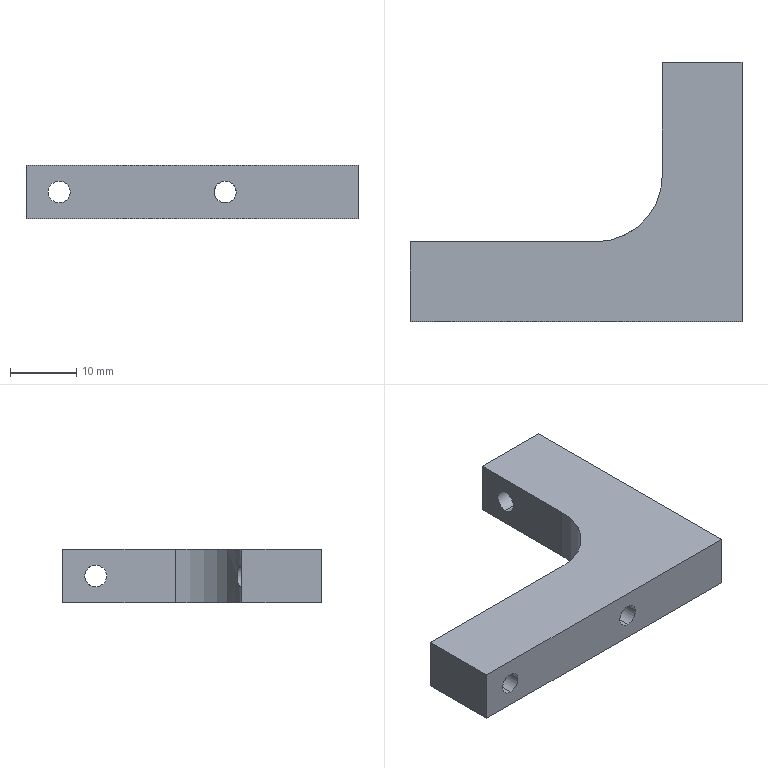CAM job | Mastercam | mm | 4 operations | part box 50 x 39 x 8
1. Drill/Counterbore | 2 - 6定位倒角
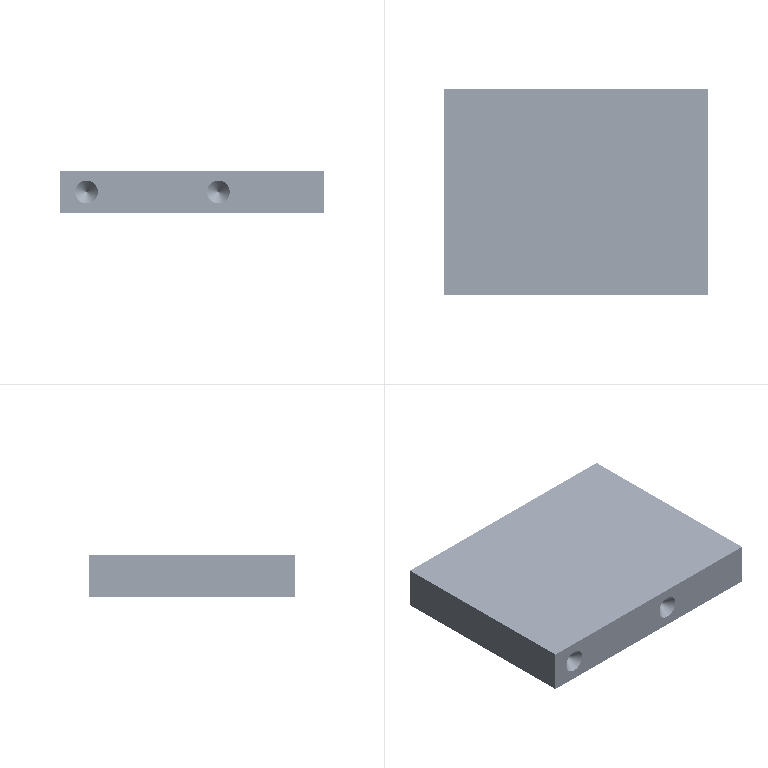2. Peck Drill | 12 - 3.3 钻头
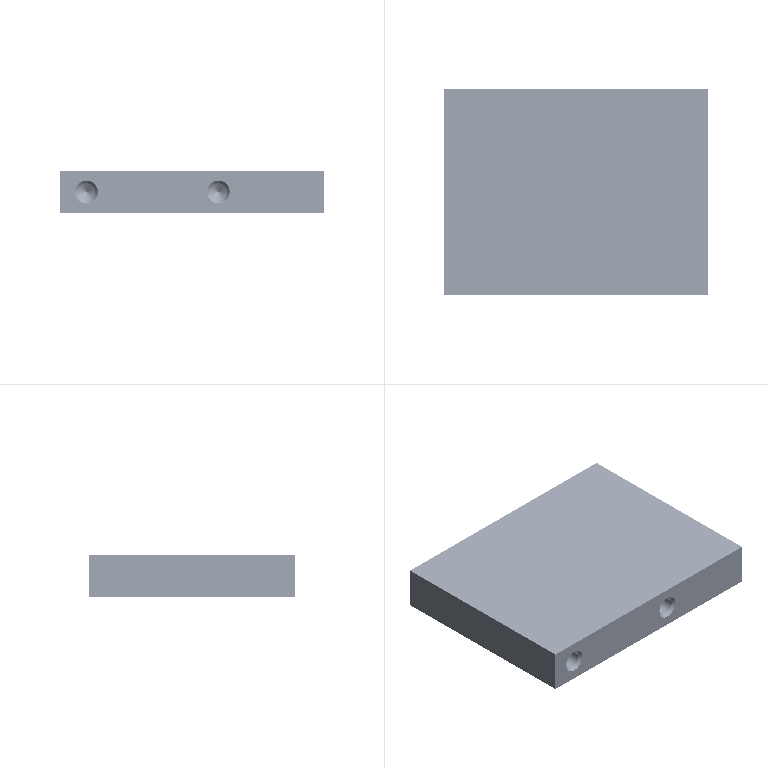3. Drill/Counterbore | 2 - 6定位倒角
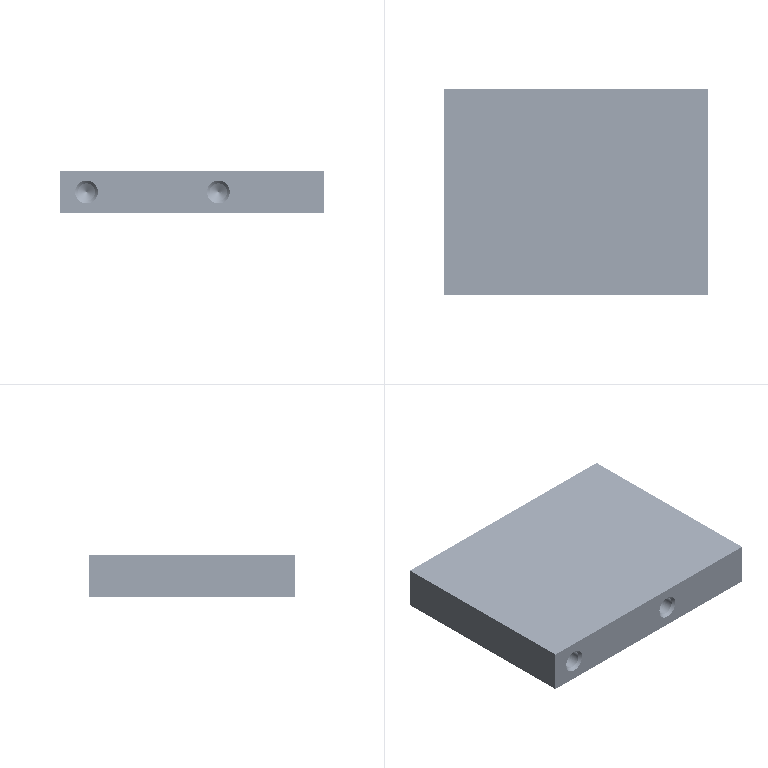4. Peck Drill | 12 - 3.3 钻头